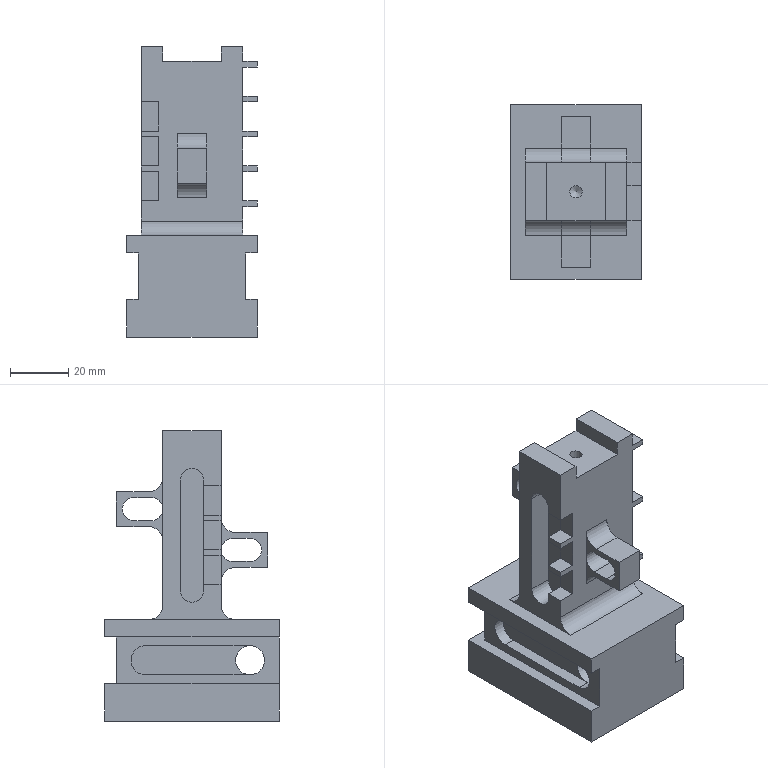Component | NX | SUPPORT_BLOCK | 1 solid | 102 faces | volume 120819 mm3 | plane 79 | cylinder 20 | cone 3 | commonest cylinder face diameters 10 x9 8 x6 4.2 x3 4.826 x2